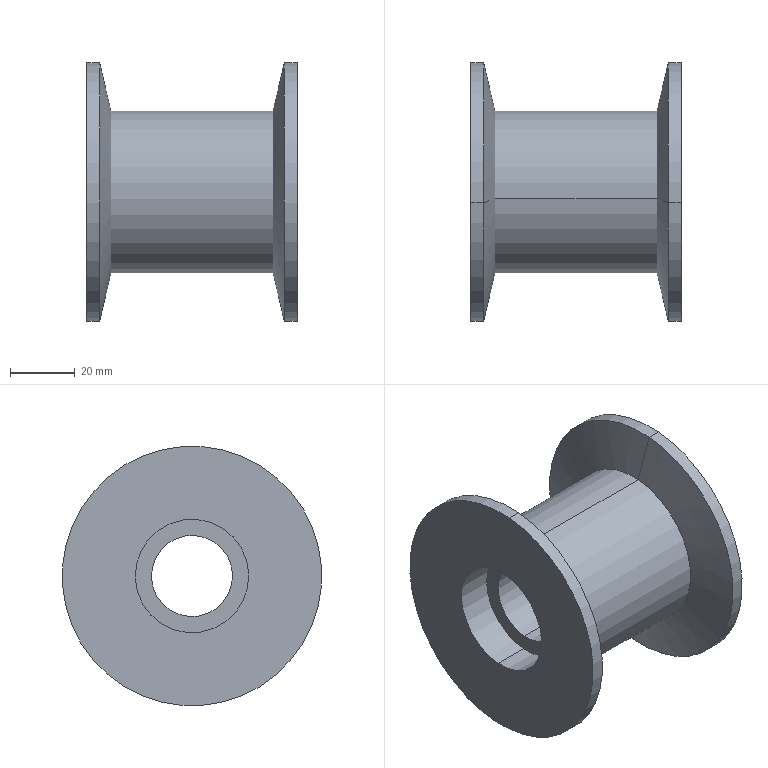Component | SolidWorks | ElectricalBoxAssembly2-1_UpperGuideWheel-1 | 1 solid | 20 faces | box 65 x 80 x 80 mm | volume 119754 mm3 | cylinder 12 | cone 4 | plane 4 | commonest cylinder face diameters 35 x4 80 x4 25 x2 50 x2
build123d program:
from build123d import *


with BuildPart() as part:
    # Sketch1 → Revolve1 (revolve)
    with BuildSketch(Plane.XY, mode=Mode.PRIVATE) as revolve1_sk:
        Polygon((0, 17.5), (0, 40), (4, 40), (7.5, 25), (57.5, 25), (61, 40), (65, 40), (65, 17.5), (54, 17.5), (54, 12.5), (11, 12.5), (11, 17.5), align=None)
    revolve(revolve1_sk.sketch.rotate(Axis((-9.535, 0, 0), (1, 0, 0)), 90), axis=Axis((-9.535, 0, 0), (1, 0, 0)))


solid = part.part

# Placed as in the assembly
solid = solid.moved(Location((653.468, -65.334, 1576.399), (0, 0, 0)))
STEP:
#1=CARTESIAN_POINT('',(27.853,-2.514,61.376));
#2=VERTEX_POINT('',#1);
#3=CARTESIAN_POINT('',(27.853,-2.631,62.749));
#4=VERTEX_POINT('',#3);
#5=CARTESIAN_POINT('',(27.853,-2.572,62.063));
#6=DIRECTION('',(1.,-0.,0.));
#7=DIRECTION('',(0.,-0.08517,0.9964));
#8=AXIS2_PLACEMENT_3D('',#5,#6,#7);
#9=CIRCLE('',#8,0.689);
#10=EDGE_CURVE('',#2,#4,#9,.T.);
#11=ORIENTED_EDGE('',*,*,#10,.F.);
#12=CARTESIAN_POINT('',(28.286,-2.514,61.376));
#13=VERTEX_POINT('',#12);
#14=CARTESIAN_POINT('',(28.662,-2.514,61.376));
#15=DIRECTION('',(1.,-0.,0.));
#16=VECTOR('',#15,39.37);
#17=LINE('',#14,#16);
#18=EDGE_CURVE('',#2,#13,#17,.T.);
#19=ORIENTED_EDGE('',*,*,#18,.T.);
#20=CARTESIAN_POINT('',(28.286,-2.631,62.749));
#21=VERTEX_POINT('',#20);
#22=CARTESIAN_POINT('',(28.286,-2.572,62.063));
#23=DIRECTION('',(1.,-0.,0.));
#24=DIRECTION('',(0.,-0.08517,0.9964));
#25=AXIS2_PLACEMENT_3D('',#22,#23,#24);
#26=CIRCLE('',#25,0.689);
#27=EDGE_CURVE('',#13,#21,#26,.T.);
#28=ORIENTED_EDGE('',*,*,#27,.T.);
#29=CARTESIAN_POINT('',(28.662,-2.631,62.749));
#30=DIRECTION('',(1.,-0.,0.));
#31=VECTOR('',#30,39.37);
#32=LINE('',#29,#31);
#33=EDGE_CURVE('',#4,#21,#32,.T.);
#34=ORIENTED_EDGE('',*,*,#33,.F.);
#35=EDGE_LOOP('',(#11,#19,#28,#34));
#36=FACE_OUTER_BOUND('',#35,.T.);
#37=CARTESIAN_POINT('',(28.662,-2.572,62.063));
#38=DIRECTION('',(1.,-0.,0.));
#39=DIRECTION('',(0.,-0.08517,0.9964));
#40=AXIS2_PLACEMENT_3D('',#37,#38,#39);
#41=CYLINDRICAL_SURFACE('',#40,0.689);
#42=ADVANCED_FACE('',(#36),#41,.F.);
#43=CARTESIAN_POINT('',(26.16,-2.53,61.573));
#44=VERTEX_POINT('',#43);
#45=CARTESIAN_POINT('',(26.16,-2.614,62.553));
#46=VERTEX_POINT('',#45);
#47=CARTESIAN_POINT('',(26.16,-2.572,62.063));
#48=DIRECTION('',(1.,-0.,0.));
#49=DIRECTION('',(0.,-0.08517,0.9964));
#50=AXIS2_PLACEMENT_3D('',#47,#48,#49);
#51=CIRCLE('',#50,0.4921);
#52=EDGE_CURVE('',#44,#46,#51,.T.);
#53=ORIENTED_EDGE('',*,*,#52,.F.);
#54=CARTESIAN_POINT('',(27.853,-2.53,61.573));
#55=VERTEX_POINT('',#54);
#56=CARTESIAN_POINT('',(28.662,-2.53,61.573));
#57=DIRECTION('',(1.,-0.,0.));
#58=VECTOR('',#57,39.37);
#59=LINE('',#56,#58);
#60=EDGE_CURVE('',#44,#55,#59,.T.);
#61=ORIENTED_EDGE('',*,*,#60,.T.);
#62=CARTESIAN_POINT('',(27.853,-2.614,62.553));
#63=VERTEX_POINT('',#62);
#64=CARTESIAN_POINT('',(27.853,-2.572,62.063));
#65=DIRECTION('',(1.,-0.,0.));
#66=DIRECTION('',(0.,-0.08517,0.9964));
#67=AXIS2_PLACEMENT_3D('',#64,#65,#66);
#68=CIRCLE('',#67,0.4921);
#69=EDGE_CURVE('',#55,#63,#68,.T.);
#70=ORIENTED_EDGE('',*,*,#69,.T.);
#71=CARTESIAN_POINT('',(28.662,-2.614,62.553));
#72=DIRECTION('',(1.,-0.,0.));
#73=VECTOR('',#72,39.37);
#74=LINE('',#71,#73);
#75=EDGE_CURVE('',#46,#63,#74,.T.);
#76=ORIENTED_EDGE('',*,*,#75,.F.);
#77=EDGE_LOOP('',(#53,#61,#70,#76));
#78=FACE_OUTER_BOUND('',#77,.T.);
#79=CARTESIAN_POINT('',(28.662,-2.572,62.063));
#80=DIRECTION('',(1.,-0.,0.));
#81=DIRECTION('',(0.,-0.08517,0.9964));
#82=AXIS2_PLACEMENT_3D('',#79,#80,#81);
#83=CYLINDRICAL_SURFACE('',#82,0.4921);
#84=ADVANCED_FACE('',(#78),#83,.F.);
#85=CARTESIAN_POINT('',(25.727,-2.514,61.376));
#86=VERTEX_POINT('',#85);
#87=CARTESIAN_POINT('',(25.727,-2.631,62.749));
#88=VERTEX_POINT('',#87);
#89=CARTESIAN_POINT('',(25.727,-2.572,62.063));
#90=DIRECTION('',(1.,-0.,0.));
#91=DIRECTION('',(0.,-0.08517,0.9964));
#92=AXIS2_PLACEMENT_3D('',#89,#90,#91);
#93=CIRCLE('',#92,0.689);
#94=EDGE_CURVE('',#86,#88,#93,.T.);
#95=ORIENTED_EDGE('',*,*,#94,.F.);
#96=CARTESIAN_POINT('',(26.16,-2.514,61.376));
#97=VERTEX_POINT('',#96);
#98=CARTESIAN_POINT('',(28.662,-2.514,61.376));
#99=DIRECTION('',(1.,-0.,0.));
#100=VECTOR('',#99,39.37);
#101=LINE('',#98,#100);
#102=EDGE_CURVE('',#86,#97,#101,.T.);
#103=ORIENTED_EDGE('',*,*,#102,.T.);
#104=CARTESIAN_POINT('',(26.16,-2.631,62.749));
#105=VERTEX_POINT('',#104);
#106=CARTESIAN_POINT('',(26.16,-2.572,62.063));
#107=DIRECTION('',(1.,-0.,0.));
#108=DIRECTION('',(0.,-0.08517,0.9964));
#109=AXIS2_PLACEMENT_3D('',#106,#107,#108);
#110=CIRCLE('',#109,0.689);
#111=EDGE_CURVE('',#97,#105,#110,.T.);
#112=ORIENTED_EDGE('',*,*,#111,.T.);
#113=CARTESIAN_POINT('',(28.662,-2.631,62.749));
#114=DIRECTION('',(1.,-0.,0.));
#115=VECTOR('',#114,39.37);
#116=LINE('',#113,#115);
#117=EDGE_CURVE('',#88,#105,#116,.T.);
#118=ORIENTED_EDGE('',*,*,#117,.F.);
#119=EDGE_LOOP('',(#95,#103,#112,#118));
#120=FACE_OUTER_BOUND('',#119,.T.);
#121=CARTESIAN_POINT('',(28.662,-2.572,62.063));
#122=DIRECTION('',(1.,-0.,0.));
#123=DIRECTION('',(0.,-0.08517,0.9964));
#124=AXIS2_PLACEMENT_3D('',#121,#122,#123);
#125=CYLINDRICAL_SURFACE('',#124,0.689);
#126=ADVANCED_FACE('',(#120),#125,.F.);
#127=CARTESIAN_POINT('',(25.727,-2.706,63.632));
#128=VERTEX_POINT('',#127);
#129=CARTESIAN_POINT('',(25.727,-2.438,60.494));
#130=VERTEX_POINT('',#129);
#131=CARTESIAN_POINT('',(25.727,-2.572,62.063));
#132=DIRECTION('',(1.,-0.,0.));
#133=DIRECTION('',(0.,-0.08517,0.9964));
#134=AXIS2_PLACEMENT_3D('',#131,#132,#133);
#135=CIRCLE('',#134,1.575);
#136=EDGE_CURVE('',#128,#130,#135,.T.);
#137=ORIENTED_EDGE('',*,*,#136,.T.);
#138=CARTESIAN_POINT('',(25.885,-2.438,60.494));
#139=VERTEX_POINT('',#138);
#140=CARTESIAN_POINT('',(28.662,-2.438,60.494));
#141=DIRECTION('',(1.,-0.,0.));
#142=VECTOR('',#141,39.37);
#143=LINE('',#140,#142);
#144=EDGE_CURVE('',#130,#139,#143,.T.);
#145=ORIENTED_EDGE('',*,*,#144,.T.);
#146=CARTESIAN_POINT('',(25.885,-2.706,63.632));
#147=VERTEX_POINT('',#146);
#148=CARTESIAN_POINT('',(25.885,-2.572,62.063));
#149=DIRECTION('',(1.,-0.,0.));
#150=DIRECTION('',(0.,-0.08517,0.9964));
#151=AXIS2_PLACEMENT_3D('',#148,#149,#150);
#152=CIRCLE('',#151,1.575);
#153=EDGE_CURVE('',#147,#139,#152,.T.);
#154=ORIENTED_EDGE('',*,*,#153,.F.);
#155=CARTESIAN_POINT('',(28.662,-2.706,63.632));
#156=DIRECTION('',(1.,-0.,0.));
#157=VECTOR('',#156,39.37);
#158=LINE('',#155,#157);
#159=EDGE_CURVE('',#128,#147,#158,.T.);
#160=ORIENTED_EDGE('',*,*,#159,.F.);
#161=EDGE_LOOP('',(#137,#145,#154,#160));
#162=FACE_OUTER_BOUND('',#161,.T.);
#163=CARTESIAN_POINT('',(28.662,-2.572,62.063));
#164=DIRECTION('',(1.,-0.,0.));
#165=DIRECTION('',(0.,-0.08517,0.9964));
#166=AXIS2_PLACEMENT_3D('',#163,#164,#165);
#167=CYLINDRICAL_SURFACE('',#166,1.575);
#168=ADVANCED_FACE('',(#162),#167,.T.);
#169=CARTESIAN_POINT('',(26.022,-2.656,63.044));
#170=VERTEX_POINT('',#169);
#171=CARTESIAN_POINT('',(26.022,-2.488,61.082));
#172=VERTEX_POINT('',#171);
#173=CARTESIAN_POINT('',(26.022,-2.572,62.063));
#174=DIRECTION('',(1.,-0.,0.));
#175=DIRECTION('',(0.,-0.08517,0.9964));
#176=AXIS2_PLACEMENT_3D('',#173,#174,#175);
#177=CIRCLE('',#176,0.9843);
#178=EDGE_CURVE('',#170,#172,#177,.T.);
#179=ORIENTED_EDGE('',*,*,#178,.F.);
#180=CARTESIAN_POINT('',(25.885,-2.706,63.632));
#181=DIRECTION('',(-0.2272,-0.08294,0.9703));
#182=VECTOR('',#181,39.37);
#183=LINE('',#180,#182);
#184=EDGE_CURVE('',#170,#147,#183,.T.);
#185=ORIENTED_EDGE('',*,*,#184,.T.);
#186=ORIENTED_EDGE('',*,*,#153,.T.);
#187=CARTESIAN_POINT('',(25.885,-2.438,60.494));
#188=DIRECTION('',(-0.2272,0.08294,-0.9703));
#189=VECTOR('',#188,39.37);
#190=LINE('',#187,#189);
#191=EDGE_CURVE('',#172,#139,#190,.T.);
#192=ORIENTED_EDGE('',*,*,#191,.F.);
#193=EDGE_LOOP('',(#179,#185,#186,#192));
#194=FACE_OUTER_BOUND('',#193,.T.);
#195=CARTESIAN_POINT('',(25.885,-2.572,62.063));
#196=DIRECTION('',(-1.,0.,-0.));
#197=DIRECTION('',(0.,0.08517,-0.9964));
#198=AXIS2_PLACEMENT_3D('',#195,#196,#197);
#199=CONICAL_SURFACE('',#198,1.575,1.342);
#200=ADVANCED_FACE('',(#194),#199,.T.);
#201=ORIENTED_EDGE('',*,*,#178,.T.);
#202=CARTESIAN_POINT('',(27.991,-2.488,61.082));
#203=VERTEX_POINT('',#202);
#204=CARTESIAN_POINT('',(28.662,-2.488,61.082));
#205=DIRECTION('',(1.,-0.,0.));
#206=VECTOR('',#205,39.37);
#207=LINE('',#204,#206);
#208=EDGE_CURVE('',#172,#203,#207,.T.);
#209=ORIENTED_EDGE('',*,*,#208,.T.);
#210=CARTESIAN_POINT('',(27.991,-2.656,63.044));
#211=VERTEX_POINT('',#210);
#212=CARTESIAN_POINT('',(27.991,-2.572,62.063));
#213=DIRECTION('',(1.,-0.,0.));
#214=DIRECTION('',(0.,-0.08517,0.9964));
#215=AXIS2_PLACEMENT_3D('',#212,#213,#214);
#216=CIRCLE('',#215,0.9843);
#217=EDGE_CURVE('',#211,#203,#216,.T.);
#218=ORIENTED_EDGE('',*,*,#217,.F.);
#219=CARTESIAN_POINT('',(28.662,-2.656,63.044));
#220=DIRECTION('',(1.,-0.,0.));
#221=VECTOR('',#220,39.37);
#222=LINE('',#219,#221);
#223=EDGE_CURVE('',#170,#211,#222,.T.);
#224=ORIENTED_EDGE('',*,*,#223,.F.);
#225=EDGE_LOOP('',(#201,#209,#218,#224));
#226=FACE_OUTER_BOUND('',#225,.T.);
#227=CARTESIAN_POINT('',(28.662,-2.572,62.063));
#228=DIRECTION('',(1.,-0.,0.));
#229=DIRECTION('',(0.,-0.08517,0.9964));
#230=AXIS2_PLACEMENT_3D('',#227,#228,#229);
#231=CYLINDRICAL_SURFACE('',#230,0.9843);
#232=ADVANCED_FACE('',(#226),#231,.T.);
#233=ORIENTED_EDGE('',*,*,#217,.T.);
#234=CARTESIAN_POINT('',(28.129,-2.438,60.494));
#235=VERTEX_POINT('',#234);
#236=CARTESIAN_POINT('',(27.991,-2.488,61.082));
#237=DIRECTION('',(0.2272,0.08294,-0.9703));
#238=VECTOR('',#237,39.37);
#239=LINE('',#236,#238);
#240=EDGE_CURVE('',#203,#235,#239,.T.);
#241=ORIENTED_EDGE('',*,*,#240,.T.);
#242=CARTESIAN_POINT('',(28.129,-2.706,63.632));
#243=VERTEX_POINT('',#242);
#244=CARTESIAN_POINT('',(28.129,-2.572,62.063));
#245=DIRECTION('',(1.,-0.,0.));
#246=DIRECTION('',(0.,-0.08517,0.9964));
#247=AXIS2_PLACEMENT_3D('',#244,#245,#246);
#248=CIRCLE('',#247,1.575);
#249=EDGE_CURVE('',#243,#235,#248,.T.);
#250=ORIENTED_EDGE('',*,*,#249,.F.);
#251=CARTESIAN_POINT('',(27.991,-2.656,63.044));
#252=DIRECTION('',(0.2272,-0.08294,0.9703));
#253=VECTOR('',#252,39.37);
#254=LINE('',#251,#253);
#255=EDGE_CURVE('',#211,#243,#254,.T.);
#256=ORIENTED_EDGE('',*,*,#255,.F.);
#257=EDGE_LOOP('',(#233,#241,#250,#256));
#258=FACE_OUTER_BOUND('',#257,.T.);
#259=CARTESIAN_POINT('',(27.991,-2.572,62.063));
#260=DIRECTION('',(1.,-0.,0.));
#261=DIRECTION('',(0.,-0.08517,0.9964));
#262=AXIS2_PLACEMENT_3D('',#259,#260,#261);
#263=CONICAL_SURFACE('',#262,0.9843,1.342);
#264=ADVANCED_FACE('',(#258),#263,.T.);
#265=ORIENTED_EDGE('',*,*,#249,.T.);
#266=CARTESIAN_POINT('',(28.286,-2.438,60.494));
#267=VERTEX_POINT('',#266);
#268=CARTESIAN_POINT('',(28.662,-2.438,60.494));
#269=DIRECTION('',(1.,-0.,0.));
#270=VECTOR('',#269,39.37);
#271=LINE('',#268,#270);
#272=EDGE_CURVE('',#235,#267,#271,.T.);
#273=ORIENTED_EDGE('',*,*,#272,.T.);
#274=CARTESIAN_POINT('',(28.286,-2.706,63.632));
#275=VERTEX_POINT('',#274);
#276=CARTESIAN_POINT('',(28.286,-2.572,62.063));
#277=DIRECTION('',(1.,-0.,0.));
#278=DIRECTION('',(0.,-0.08517,0.9964));
#279=AXIS2_PLACEMENT_3D('',#276,#277,#278);
#280=CIRCLE('',#279,1.575);
#281=EDGE_CURVE('',#275,#267,#280,.T.);
#282=ORIENTED_EDGE('',*,*,#281,.F.);
#283=CARTESIAN_POINT('',(28.662,-2.706,63.632));
#284=DIRECTION('',(1.,-0.,0.));
#285=VECTOR('',#284,39.37);
#286=LINE('',#283,#285);
#287=EDGE_CURVE('',#243,#275,#286,.T.);
#288=ORIENTED_EDGE('',*,*,#287,.F.);
#289=EDGE_LOOP('',(#265,#273,#282,#288));
#290=FACE_OUTER_BOUND('',#289,.T.);
#291=CARTESIAN_POINT('',(28.662,-2.572,62.063));
#292=DIRECTION('',(1.,-0.,0.));
#293=DIRECTION('',(0.,-0.08517,0.9964));
#294=AXIS2_PLACEMENT_3D('',#291,#292,#293);
#295=CYLINDRICAL_SURFACE('',#294,1.575);
#296=ADVANCED_FACE('',(#290),#295,.T.);
#297=ORIENTED_EDGE('',*,*,#272,.F.);
#298=CARTESIAN_POINT('',(28.129,-2.572,62.063));
#299=DIRECTION('',(1.,-0.,0.));
#300=DIRECTION('',(0.,-0.08517,0.9964));
#301=AXIS2_PLACEMENT_3D('',#298,#299,#300);
#302=CIRCLE('',#301,1.575);
#303=EDGE_CURVE('',#235,#243,#302,.T.);
#304=ORIENTED_EDGE('',*,*,#303,.T.);
#305=ORIENTED_EDGE('',*,*,#287,.T.);
#306=CARTESIAN_POINT('',(28.286,-2.572,62.063));
#307=DIRECTION('',(1.,-0.,0.));
#308=DIRECTION('',(0.,-0.08517,0.9964));
#309=AXIS2_PLACEMENT_3D('',#306,#307,#308);
#310=CIRCLE('',#309,1.575);
#311=EDGE_CURVE('',#267,#275,#310,.T.);
#312=ORIENTED_EDGE('',*,*,#311,.F.);
#313=EDGE_LOOP('',(#297,#304,#305,#312));
#314=FACE_OUTER_BOUND('',#313,.T.);
#315=CARTESIAN_POINT('',(28.662,-2.572,62.063));
#316=DIRECTION('',(1.,-0.,0.));
#317=DIRECTION('',(0.,-0.08517,0.9964));
#318=AXIS2_PLACEMENT_3D('',#315,#316,#317);
#319=CYLINDRICAL_SURFACE('',#318,1.575);
#320=ADVANCED_FACE('',(#314),#319,.T.);
#321=ORIENTED_EDGE('',*,*,#240,.F.);
#322=CARTESIAN_POINT('',(27.991,-2.572,62.063));
#323=DIRECTION('',(1.,-0.,0.));
#324=DIRECTION('',(0.,-0.08517,0.9964));
#325=AXIS2_PLACEMENT_3D('',#322,#323,#324);
#326=CIRCLE('',#325,0.9843);
#327=EDGE_CURVE('',#203,#211,#326,.T.);
#328=ORIENTED_EDGE('',*,*,#327,.T.);
#329=ORIENTED_EDGE('',*,*,#255,.T.);
#330=ORIENTED_EDGE('',*,*,#303,.F.);
#331=EDGE_LOOP('',(#321,#328,#329,#330));
#332=FACE_OUTER_BOUND('',#331,.T.);
#333=CARTESIAN_POINT('',(27.991,-2.572,62.063));
#334=DIRECTION('',(1.,-0.,0.));
#335=DIRECTION('',(0.,-0.08517,0.9964));
#336=AXIS2_PLACEMENT_3D('',#333,#334,#335);
#337=CONICAL_SURFACE('',#336,0.9843,1.342);
#338=ADVANCED_FACE('',(#332),#337,.T.);
#339=ORIENTED_EDGE('',*,*,#208,.F.);
#340=CARTESIAN_POINT('',(26.022,-2.572,62.063));
#341=DIRECTION('',(1.,-0.,0.));
#342=DIRECTION('',(0.,-0.08517,0.9964));
#343=AXIS2_PLACEMENT_3D('',#340,#341,#342);
#344=CIRCLE('',#343,0.9843);
#345=EDGE_CURVE('',#172,#170,#344,.T.);
#346=ORIENTED_EDGE('',*,*,#345,.T.);
#347=ORIENTED_EDGE('',*,*,#223,.T.);
#348=ORIENTED_EDGE('',*,*,#327,.F.);
#349=EDGE_LOOP('',(#339,#346,#347,#348));
#350=FACE_OUTER_BOUND('',#349,.T.);
#351=CARTESIAN_POINT('',(28.662,-2.572,62.063));
#352=DIRECTION('',(1.,-0.,0.));
#353=DIRECTION('',(0.,-0.08517,0.9964));
#354=AXIS2_PLACEMENT_3D('',#351,#352,#353);
#355=CYLINDRICAL_SURFACE('',#354,0.9843);
#356=ADVANCED_FACE('',(#350),#355,.T.);
#357=ORIENTED_EDGE('',*,*,#184,.F.);
#358=ORIENTED_EDGE('',*,*,#345,.F.);
#359=ORIENTED_EDGE('',*,*,#191,.T.);
#360=CARTESIAN_POINT('',(25.885,-2.572,62.063));
#361=DIRECTION('',(1.,-0.,0.));
#362=DIRECTION('',(0.,-0.08517,0.9964));
#363=AXIS2_PLACEMENT_3D('',#360,#361,#362);
#364=CIRCLE('',#363,1.575);
#365=EDGE_CURVE('',#139,#147,#364,.T.);
#366=ORIENTED_EDGE('',*,*,#365,.T.);
#367=EDGE_LOOP('',(#357,#358,#359,#366));
#368=FACE_OUTER_BOUND('',#367,.T.);
#369=CARTESIAN_POINT('',(25.885,-2.572,62.063));
#370=DIRECTION('',(-1.,0.,-0.));
#371=DIRECTION('',(0.,0.08517,-0.9964));
#372=AXIS2_PLACEMENT_3D('',#369,#370,#371);
#373=CONICAL_SURFACE('',#372,1.575,1.342);
#374=ADVANCED_FACE('',(#368),#373,.T.);
#375=ORIENTED_EDGE('',*,*,#144,.F.);
#376=CARTESIAN_POINT('',(25.727,-2.572,62.063));
#377=DIRECTION('',(1.,-0.,0.));
#378=DIRECTION('',(0.,-0.08517,0.9964));
#379=AXIS2_PLACEMENT_3D('',#376,#377,#378);
#380=CIRCLE('',#379,1.575);
#381=EDGE_CURVE('',#130,#128,#380,.T.);
#382=ORIENTED_EDGE('',*,*,#381,.T.);
#383=ORIENTED_EDGE('',*,*,#159,.T.);
#384=ORIENTED_EDGE('',*,*,#365,.F.);
#385=EDGE_LOOP('',(#375,#382,#383,#384));
#386=FACE_OUTER_BOUND('',#385,.T.);
#387=CARTESIAN_POINT('',(28.662,-2.572,62.063));
#388=DIRECTION('',(1.,-0.,0.));
#389=DIRECTION('',(0.,-0.08517,0.9964));
#390=AXIS2_PLACEMENT_3D('',#387,#388,#389);
#391=CYLINDRICAL_SURFACE('',#390,1.575);
#392=ADVANCED_FACE('',(#386),#391,.T.);
#393=ORIENTED_EDGE('',*,*,#136,.F.);
#394=ORIENTED_EDGE('',*,*,#381,.F.);
#395=EDGE_LOOP('',(#393,#394));
#396=FACE_OUTER_BOUND('',#395,.T.);
#397=CARTESIAN_POINT('',(25.727,-2.572,62.063));
#398=DIRECTION('',(1.,-0.,0.));
#399=DIRECTION('',(0.,-0.08517,0.9964));
#400=AXIS2_PLACEMENT_3D('',#397,#398,#399);
#401=CIRCLE('',#400,0.689);
#402=EDGE_CURVE('',#88,#86,#401,.T.);
#403=ORIENTED_EDGE('',*,*,#402,.T.);
#404=ORIENTED_EDGE('',*,*,#94,.T.);
#405=EDGE_LOOP('',(#403,#404));
#406=FACE_BOUND('',#405,.T.);
#407=CARTESIAN_POINT('',(25.727,-4.141,61.929));
#408=DIRECTION('',(1.,-0.,0.));
#409=DIRECTION('',(-0.,-0.08517,0.9964));
#410=AXIS2_PLACEMENT_3D('',#407,#408,#409);
#411=PLANE('',#410);
#412=ADVANCED_FACE('',(#396,#406),#411,.F.);
#413=ORIENTED_EDGE('',*,*,#102,.F.);
#414=ORIENTED_EDGE('',*,*,#402,.F.);
#415=ORIENTED_EDGE('',*,*,#117,.T.);
#416=CARTESIAN_POINT('',(26.16,-2.572,62.063));
#417=DIRECTION('',(1.,-0.,0.));
#418=DIRECTION('',(0.,-0.08517,0.9964));
#419=AXIS2_PLACEMENT_3D('',#416,#417,#418);
#420=CIRCLE('',#419,0.689);
#421=EDGE_CURVE('',#105,#97,#420,.T.);
#422=ORIENTED_EDGE('',*,*,#421,.T.);
#423=EDGE_LOOP('',(#413,#414,#415,#422));
#424=FACE_OUTER_BOUND('',#423,.T.);
#425=CARTESIAN_POINT('',(28.662,-2.572,62.063));
#426=DIRECTION('',(1.,-0.,0.));
#427=DIRECTION('',(0.,-0.08517,0.9964));
#428=AXIS2_PLACEMENT_3D('',#425,#426,#427);
#429=CYLINDRICAL_SURFACE('',#428,0.689);
#430=ADVANCED_FACE('',(#424),#429,.F.);
#431=ORIENTED_EDGE('',*,*,#421,.F.);
#432=ORIENTED_EDGE('',*,*,#111,.F.);
#433=EDGE_LOOP('',(#431,#432));
#434=FACE_OUTER_BOUND('',#433,.T.);
#435=CARTESIAN_POINT('',(26.16,-2.572,62.063));
#436=DIRECTION('',(1.,-0.,0.));
#437=DIRECTION('',(0.,-0.08517,0.9964));
#438=AXIS2_PLACEMENT_3D('',#435,#436,#437);
#439=CIRCLE('',#438,0.4921);
#440=EDGE_CURVE('',#46,#44,#439,.T.);
#441=ORIENTED_EDGE('',*,*,#440,.T.);
#442=ORIENTED_EDGE('',*,*,#52,.T.);
#443=EDGE_LOOP('',(#441,#442));
#444=FACE_BOUND('',#443,.T.);
#445=CARTESIAN_POINT('',(26.16,-3.063,62.021));
#446=DIRECTION('',(1.,-0.,0.));
#447=DIRECTION('',(-0.,-0.08517,0.9964));
#448=AXIS2_PLACEMENT_3D('',#445,#446,#447);
#449=PLANE('',#448);
#450=ADVANCED_FACE('',(#434,#444),#449,.F.);
#451=ORIENTED_EDGE('',*,*,#60,.F.);
#452=ORIENTED_EDGE('',*,*,#440,.F.);
#453=ORIENTED_EDGE('',*,*,#75,.T.);
#454=CARTESIAN_POINT('',(27.853,-2.572,62.063));
#455=DIRECTION('',(1.,-0.,0.));
#456=DIRECTION('',(0.,-0.08517,0.9964));
#457=AXIS2_PLACEMENT_3D('',#454,#455,#456);
#458=CIRCLE('',#457,0.4921);
#459=EDGE_CURVE('',#63,#55,#458,.T.);
#460=ORIENTED_EDGE('',*,*,#459,.T.);
#461=EDGE_LOOP('',(#451,#452,#453,#460));
#462=FACE_OUTER_BOUND('',#461,.T.);
#463=CARTESIAN_POINT('',(28.662,-2.572,62.063));
#464=DIRECTION('',(1.,-0.,0.));
#465=DIRECTION('',(0.,-0.08517,0.9964));
#466=AXIS2_PLACEMENT_3D('',#463,#464,#465);
#467=CYLINDRICAL_SURFACE('',#466,0.4921);
#468=ADVANCED_FACE('',(#462),#467,.F.);
#469=ORIENTED_EDGE('',*,*,#459,.F.);
#470=ORIENTED_EDGE('',*,*,#69,.F.);
#471=EDGE_LOOP('',(#469,#470));
#472=FACE_BOUND('',#471,.T.);
#473=CARTESIAN_POINT('',(27.853,-2.572,62.063));
#474=DIRECTION('',(1.,-0.,0.));
#475=DIRECTION('',(0.,-0.08517,0.9964));
#476=AXIS2_PLACEMENT_3D('',#473,#474,#475);
#477=CIRCLE('',#476,0.689);
#478=EDGE_CURVE('',#4,#2,#477,.T.);
#479=ORIENTED_EDGE('',*,*,#478,.T.);
#480=ORIENTED_EDGE('',*,*,#10,.T.);
#481=EDGE_LOOP('',(#479,#480));
#482=FACE_OUTER_BOUND('',#481,.T.);
#483=CARTESIAN_POINT('',(27.853,-3.259,62.004));
#484=DIRECTION('',(-1.,0.,-0.));
#485=DIRECTION('',(0.,0.08517,-0.9964));
#486=AXIS2_PLACEMENT_3D('',#483,#484,#485);
#487=PLANE('',#486);
#488=ADVANCED_FACE('',(#472,#482),#487,.F.);
#489=ORIENTED_EDGE('',*,*,#18,.F.);
#490=ORIENTED_EDGE('',*,*,#478,.F.);
#491=ORIENTED_EDGE('',*,*,#33,.T.);
#492=CARTESIAN_POINT('',(28.286,-2.572,62.063));
#493=DIRECTION('',(1.,-0.,0.));
#494=DIRECTION('',(0.,-0.08517,0.9964));
#495=AXIS2_PLACEMENT_3D('',#492,#493,#494);
#496=CIRCLE('',#495,0.689);
#497=EDGE_CURVE('',#21,#13,#496,.T.);
#498=ORIENTED_EDGE('',*,*,#497,.T.);
#499=EDGE_LOOP('',(#489,#490,#491,#498));
#500=FACE_OUTER_BOUND('',#499,.T.);
#501=CARTESIAN_POINT('',(28.662,-2.572,62.063));
#502=DIRECTION('',(1.,-0.,0.));
#503=DIRECTION('',(0.,-0.08517,0.9964));
#504=AXIS2_PLACEMENT_3D('',#501,#502,#503);
#505=CYLINDRICAL_SURFACE('',#504,0.689);
#506=ADVANCED_FACE('',(#500),#505,.F.);
#507=ORIENTED_EDGE('',*,*,#497,.F.);
#508=ORIENTED_EDGE('',*,*,#27,.F.);
#509=EDGE_LOOP('',(#507,#508));
#510=FACE_BOUND('',#509,.T.);
#511=ORIENTED_EDGE('',*,*,#281,.T.);
#512=ORIENTED_EDGE('',*,*,#311,.T.);
#513=EDGE_LOOP('',(#511,#512));
#514=FACE_OUTER_BOUND('',#513,.T.);
#515=CARTESIAN_POINT('',(28.286,-3.259,62.004));
#516=DIRECTION('',(-1.,0.,-0.));
#517=DIRECTION('',(0.,0.08517,-0.9964));
#518=AXIS2_PLACEMENT_3D('',#515,#516,#517);
#519=PLANE('',#518);
#520=ADVANCED_FACE('',(#510,#514),#519,.F.);
#521=CLOSED_SHELL('',(#42,#84,#126,#168,#200,#232,#264,#296,#320,#338,#356,#374,#392,#412,#430,#450,#468,#488,#506,#520));
#522=MANIFOLD_SOLID_BREP('',#521);
#523=CARTESIAN_POINT('',(0.,0.,0.));
#524=DIRECTION('',(0.,0.,1.));
#525=DIRECTION('',(1.,0.,0.));
#526=AXIS2_PLACEMENT_3D('',#523,#524,#525);
#527=(LENGTH_UNIT()NAMED_UNIT(*)SI_UNIT($,.METRE.));
#528=LENGTH_MEASURE_WITH_UNIT(LENGTH_MEASURE(0.0254),#527);
#529=DIMENSIONAL_EXPONENTS(1.,0.,0.,0.,0.,0.,0.);
#530=(CONVERSION_BASED_UNIT('',#528)LENGTH_UNIT()NAMED_UNIT(#529));
#531=UNCERTAINTY_MEASURE_WITH_UNIT(LENGTH_MEASURE(0.00001),#530,'','');
#532=(NAMED_UNIT(*)PLANE_ANGLE_UNIT()SI_UNIT($,.RADIAN.));
#533=(NAMED_UNIT(*)SI_UNIT($,.STERADIAN.)SOLID_ANGLE_UNIT());
#534=(GEOMETRIC_REPRESENTATION_CONTEXT(3)GLOBAL_UNCERTAINTY_ASSIGNED_CONTEXT((#531))GLOBAL_UNIT_ASSIGNED_CONTEXT((#530,#532,#533))REPRESENTATION_CONTEXT('',''));
#535=ADVANCED_BREP_SHAPE_REPRESENTATION('',(#522,#526),#534);
#536=COLOUR_RGB('',0.7922,0.8196,0.9333);
#537=FILL_AREA_STYLE_COLOUR('',#536);
#538=FILL_AREA_STYLE('',(#537));
#539=SURFACE_STYLE_FILL_AREA(#538);
#540=SURFACE_SIDE_STYLE('',(#539));
#541=SURFACE_STYLE_USAGE(.BOTH.,#540);
#542=PRESENTATION_STYLE_ASSIGNMENT((#541));
#543=STYLED_ITEM('',(#542),#522);
#544=PRESENTATION_LAYER_ASSIGNMENT('','',(#543));
#545=(LENGTH_UNIT()NAMED_UNIT(*)SI_UNIT($,.METRE.));
#546=LENGTH_MEASURE_WITH_UNIT(LENGTH_MEASURE(0.0254),#545);
#547=DIMENSIONAL_EXPONENTS(1.,0.,0.,0.,0.,0.,0.);
#548=(CONVERSION_BASED_UNIT('',#546)LENGTH_UNIT()NAMED_UNIT(#547));
#549=UNCERTAINTY_MEASURE_WITH_UNIT(LENGTH_MEASURE(0.00001),#548,'','');
#550=(NAMED_UNIT(*)PLANE_ANGLE_UNIT()SI_UNIT($,.RADIAN.));
#551=(NAMED_UNIT(*)SI_UNIT($,.STERADIAN.)SOLID_ANGLE_UNIT());
#552=(GEOMETRIC_REPRESENTATION_CONTEXT(3)GLOBAL_UNCERTAINTY_ASSIGNED_CONTEXT((#549))GLOBAL_UNIT_ASSIGNED_CONTEXT((#548,#550,#551))REPRESENTATION_CONTEXT('',''));
#553=MECHANICAL_DESIGN_GEOMETRIC_PRESENTATION_REPRESENTATION('',(#543),#552);